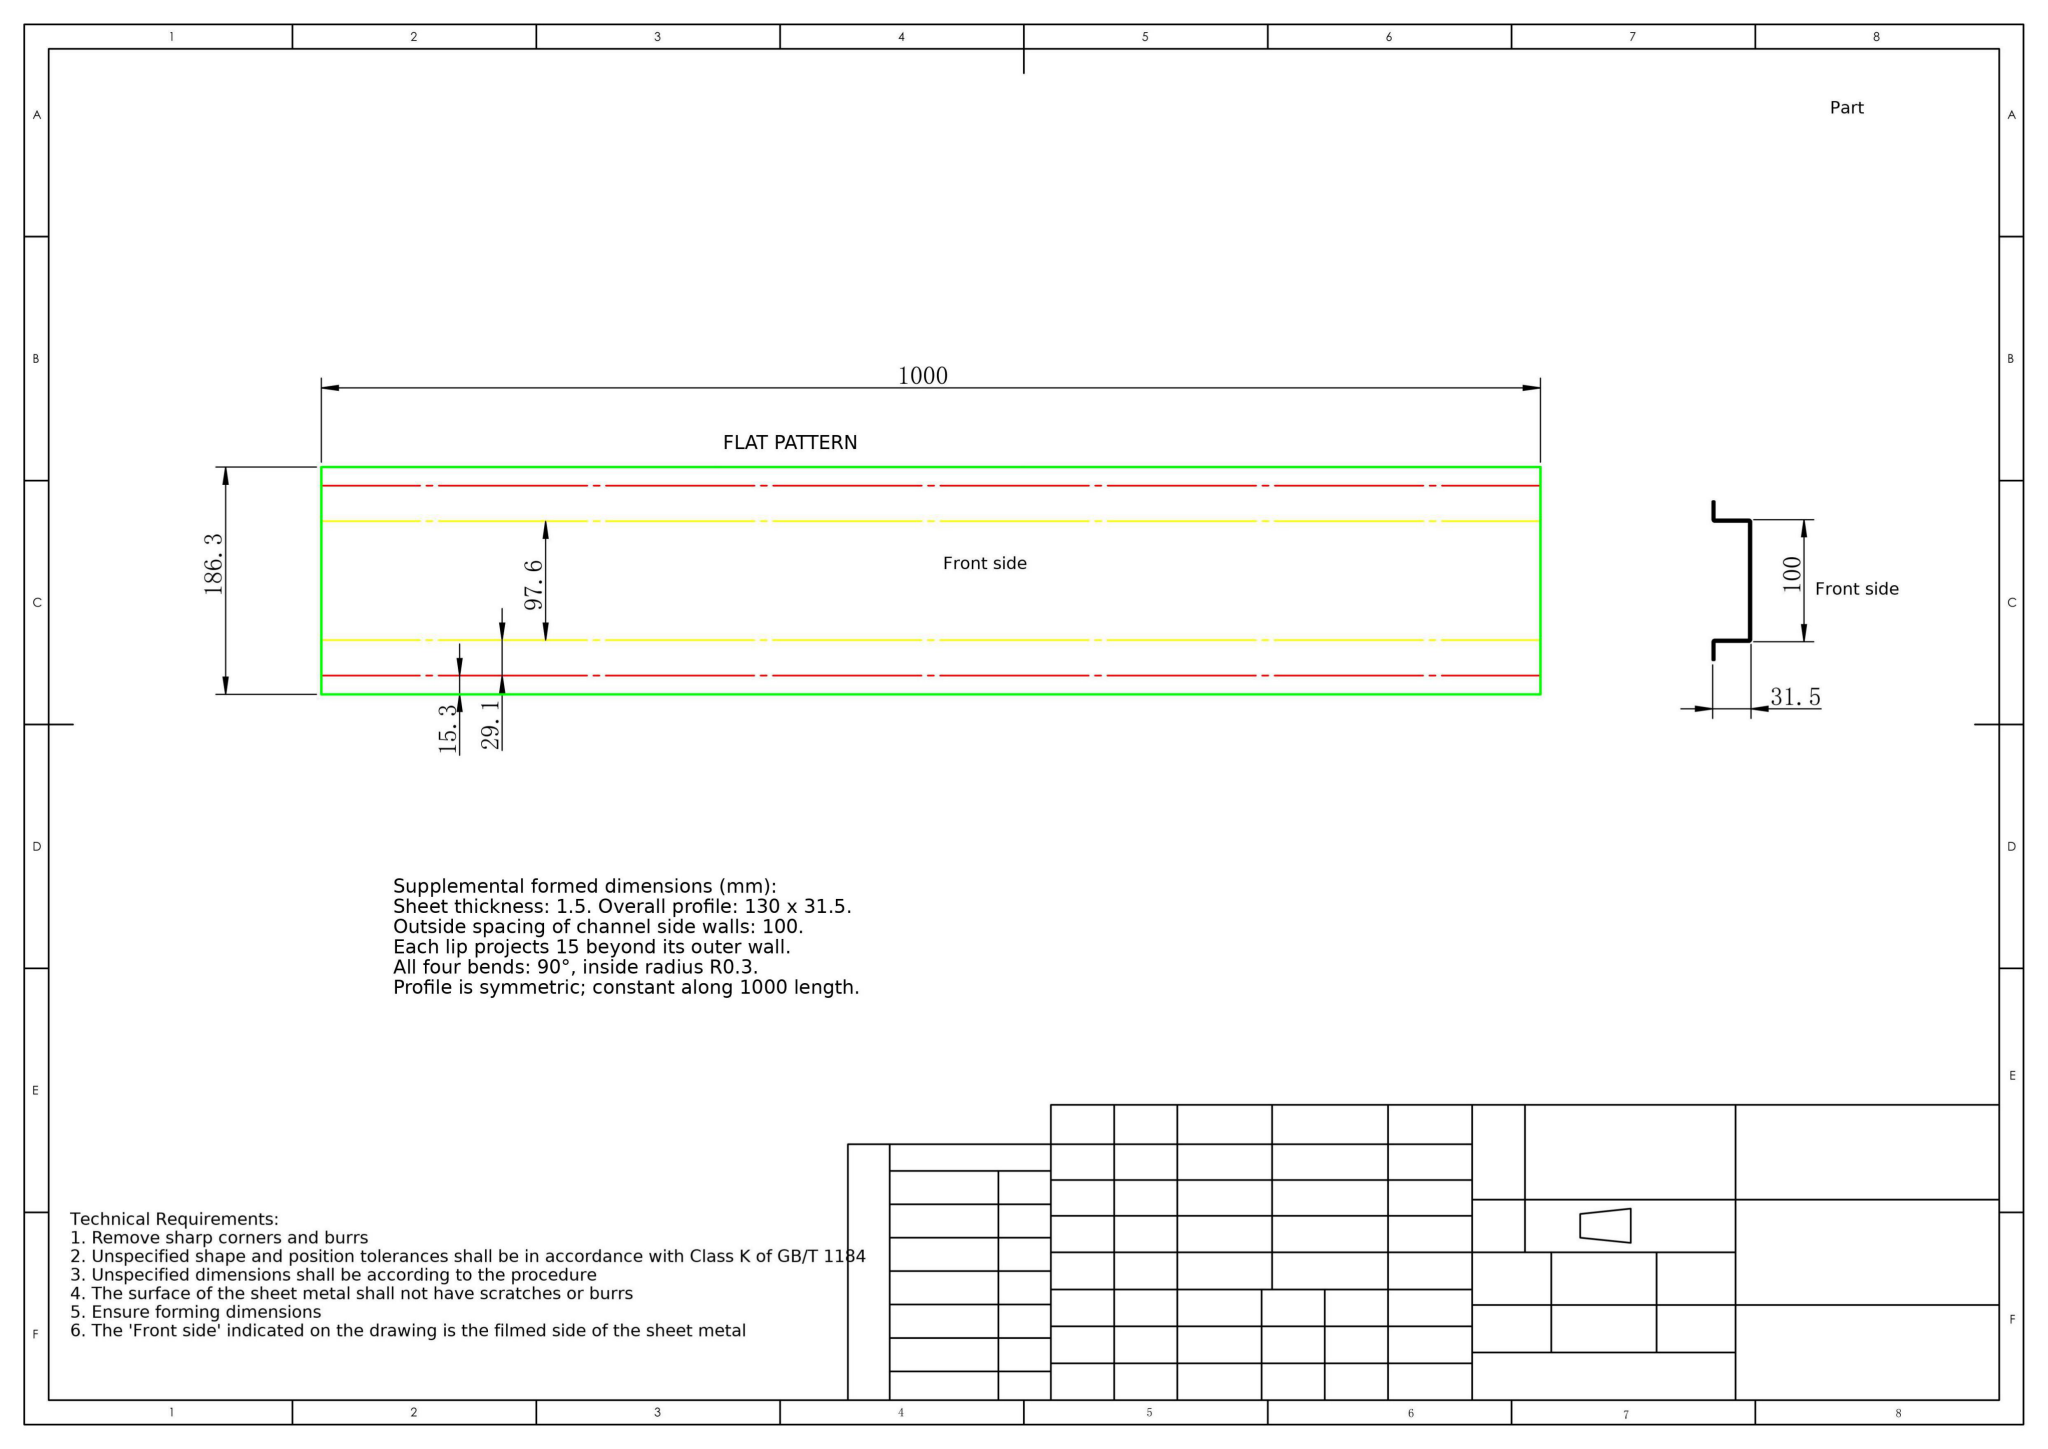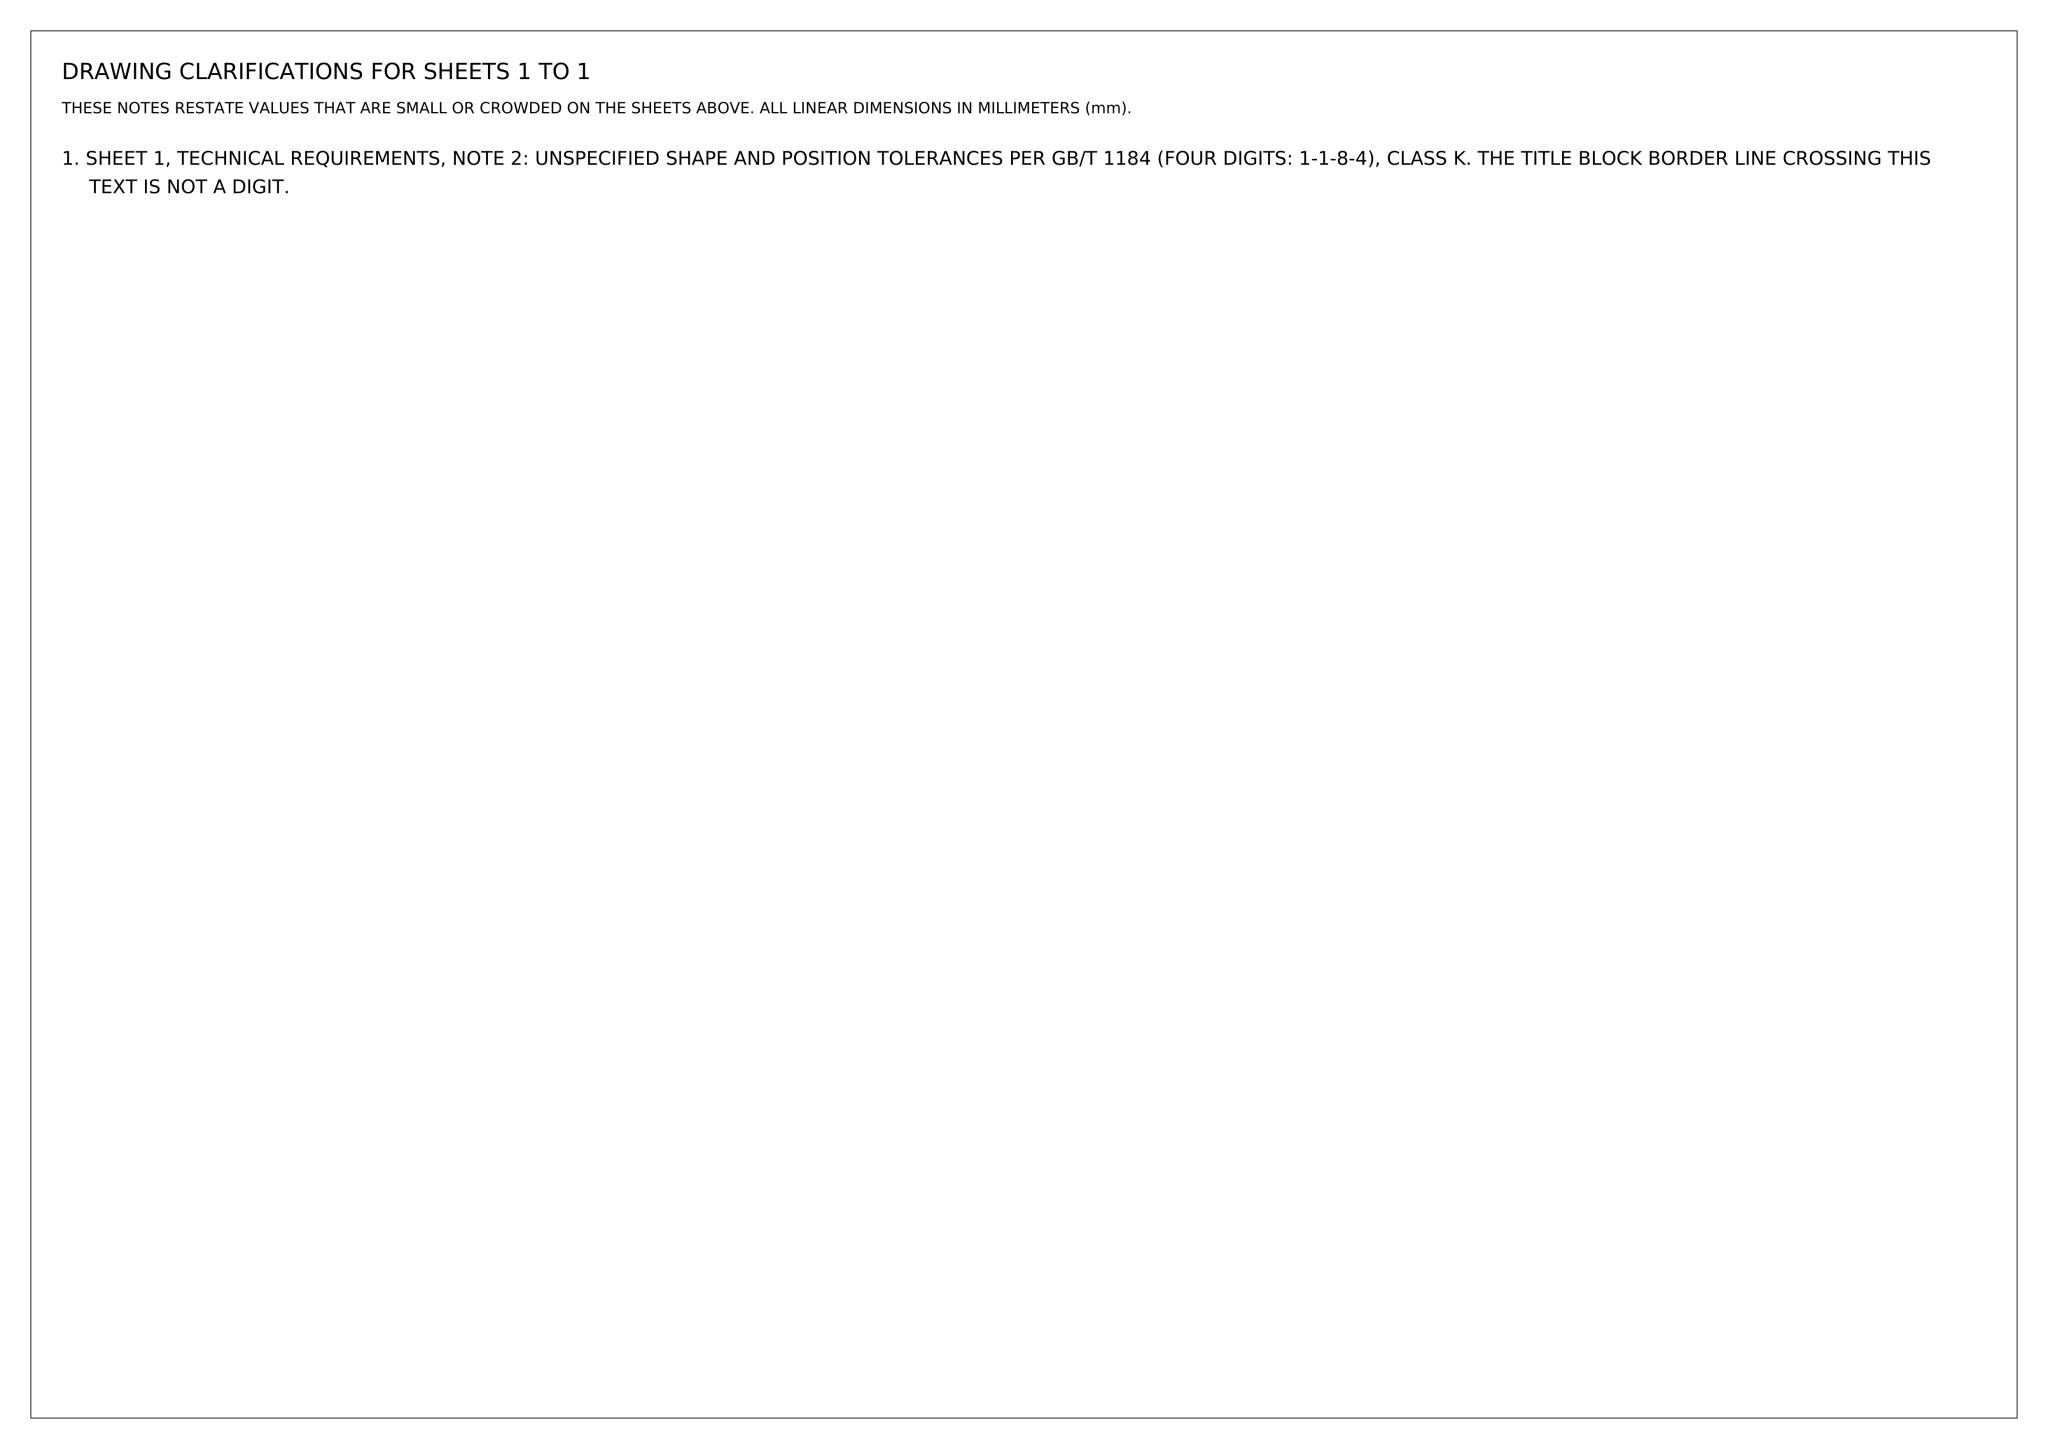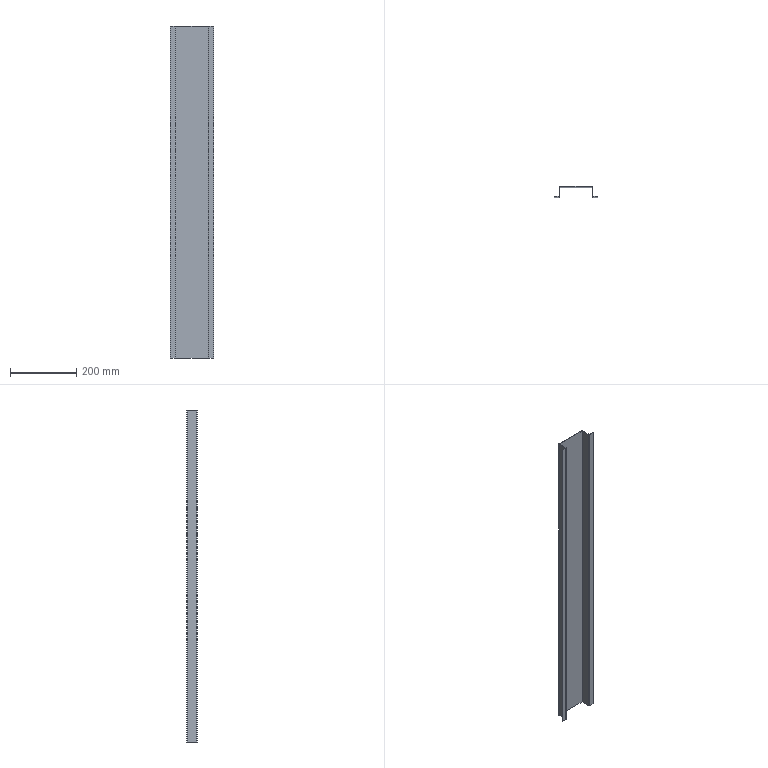Part | NX | mm | Stepped L-Channel Trim Extrusion | 1 solid | 38 faces | box 130 x 31.5 x 1000 mm | volume 282296 mm3 | plane 30 | cylinder 8 | commonest cylinder face diameters 0.6 x4 3.6 x4